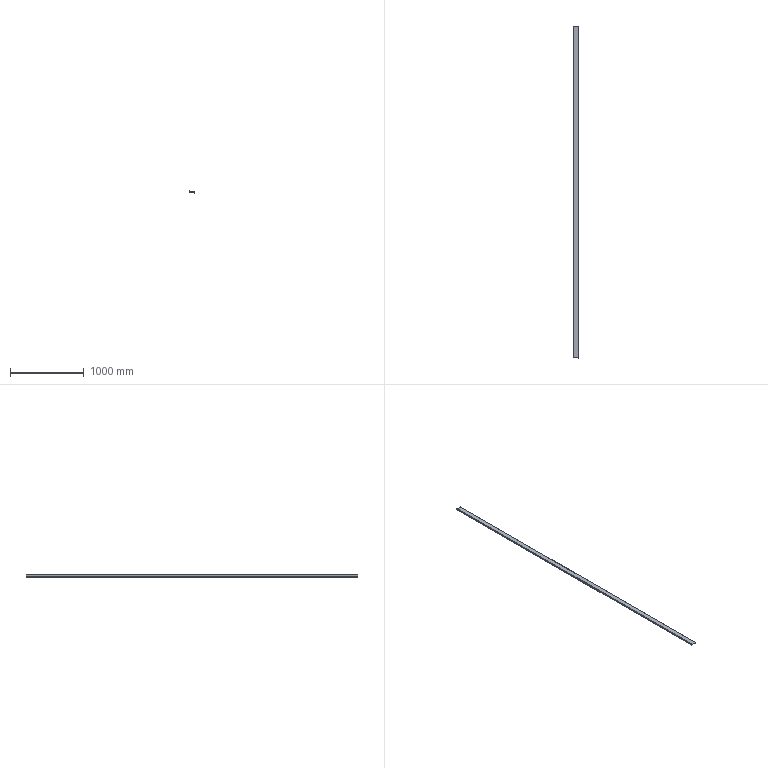Component | NX | 35_10 | 1 solid | 10 faces | volume 789750 mm3 | plane 10